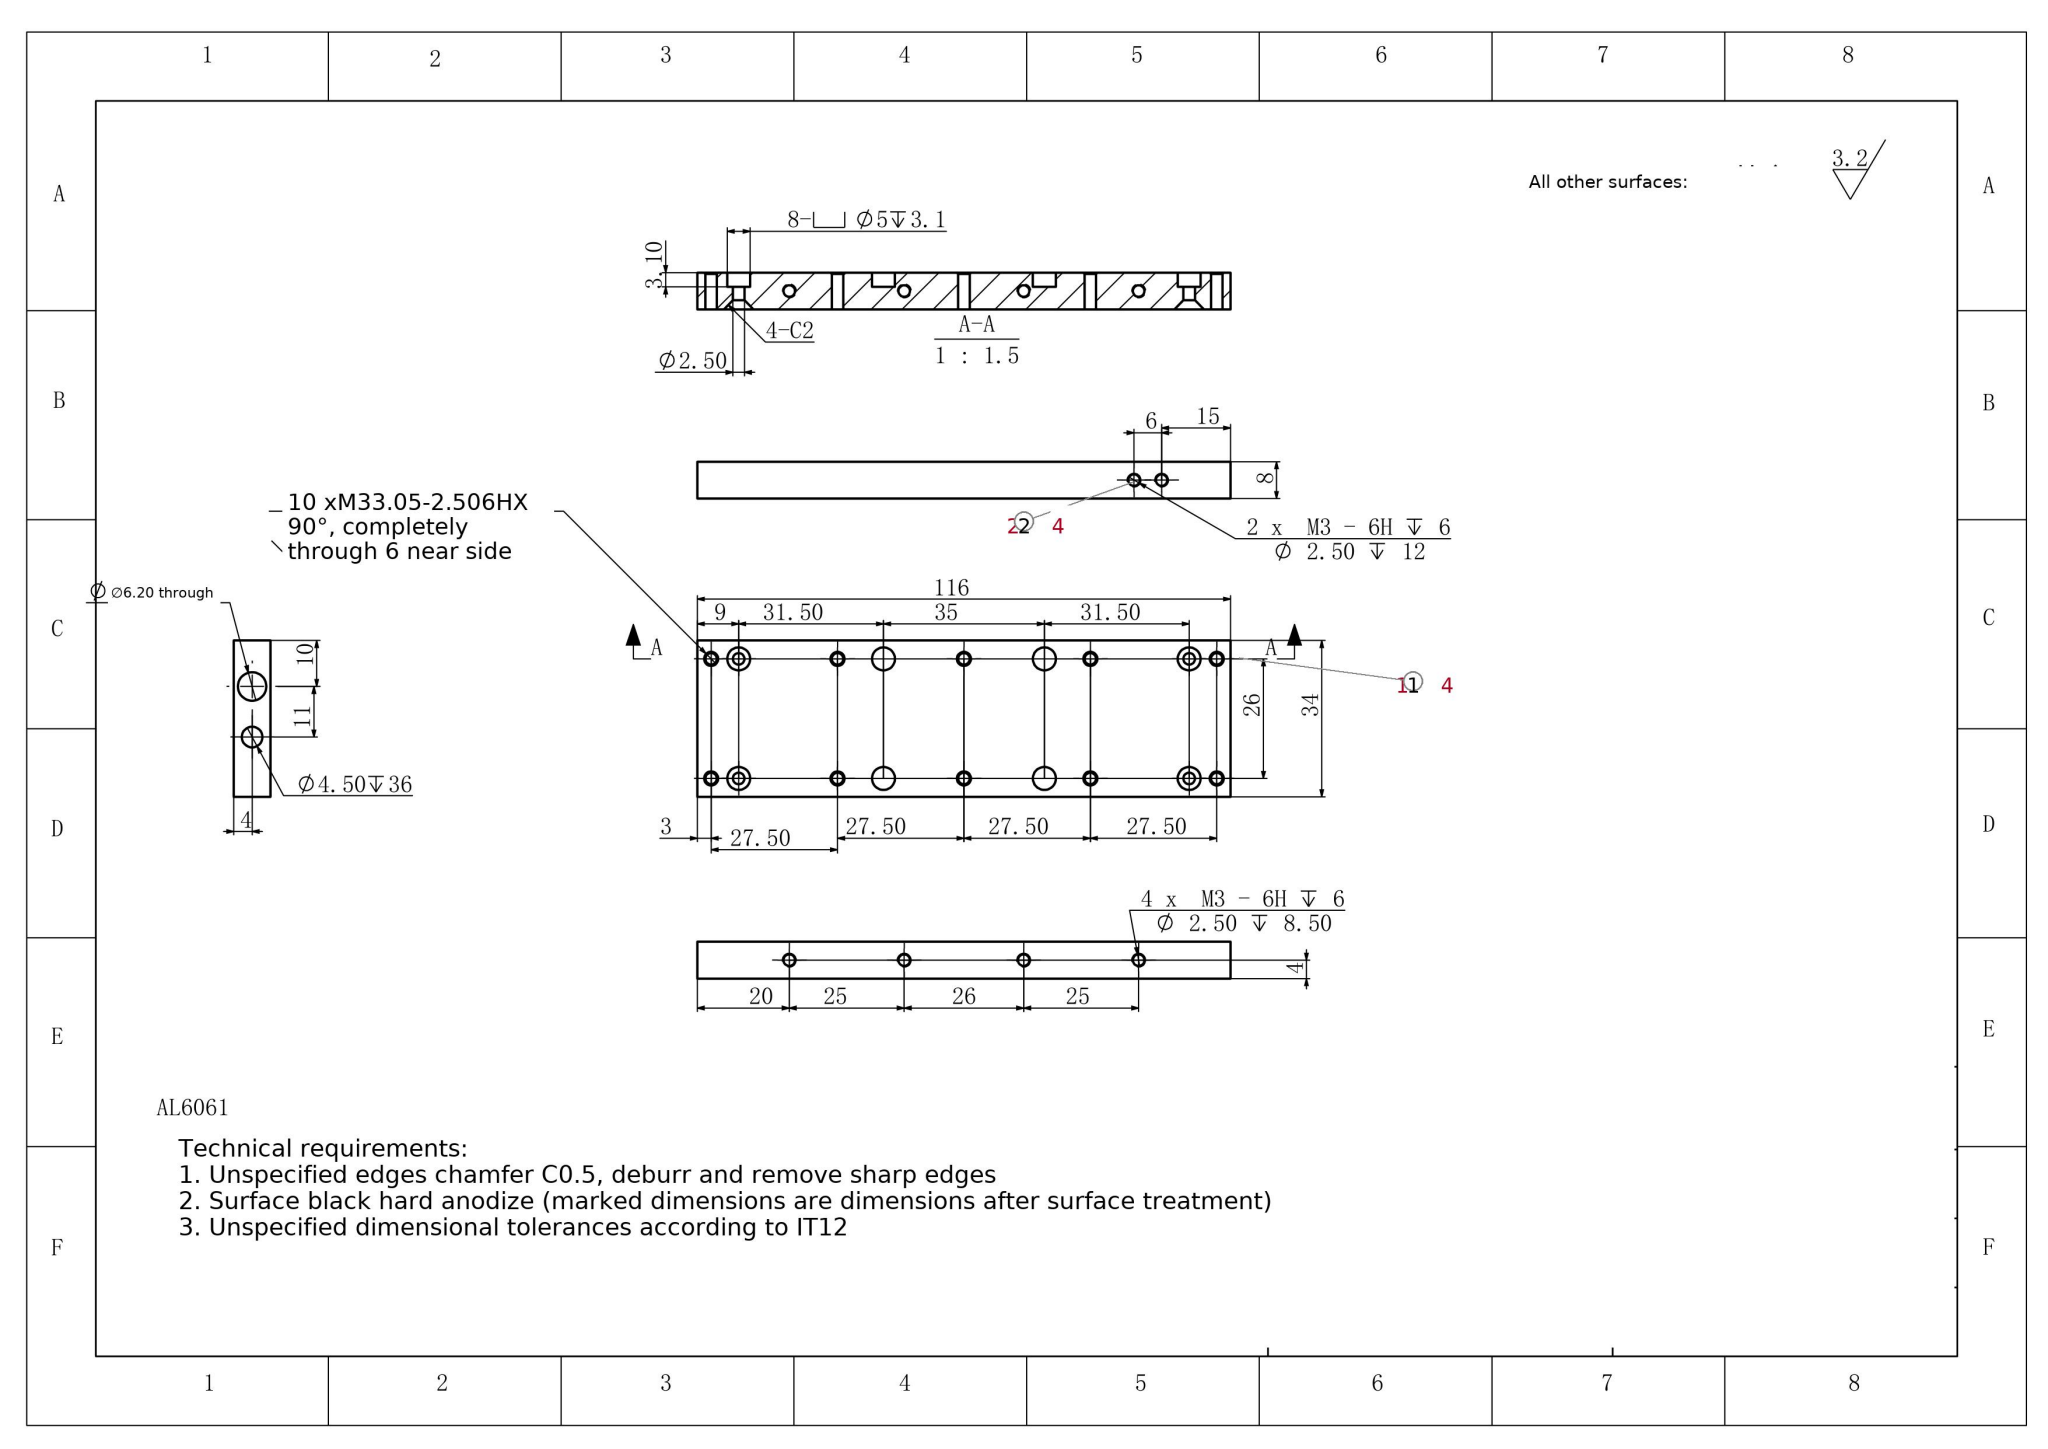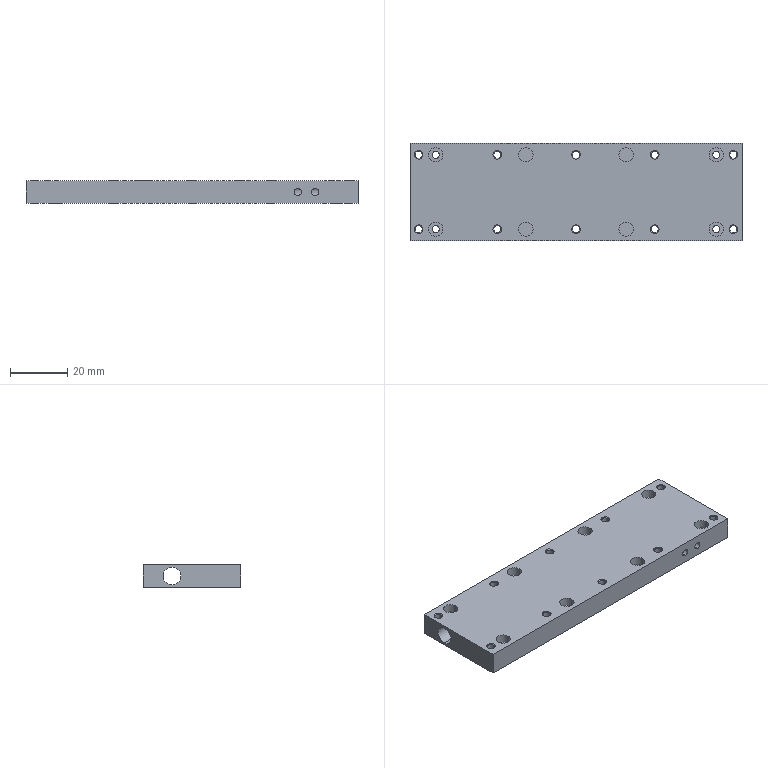Part | SolidWorks | mm | material AL6061 | 1 solid | 103 faces | box 116 x 34 x 8 mm | volume 26159 mm3 | cylinder 60 | cone 28 | plane 15 | commonest cylinder face diameters 2.5 x40 5 x16 4.5 x2 6.2 x2
build123d program:
from build123d import *

# Parameters (mm, degrees)
SKETCH1_W                   = 116
SKETCH1_H                   = 34
BOSS_EXTRUDE1_DEPTH         = 8
F_2_5_2_5_DIAMETER_HOLE1_D  = 2.5
M3_TAPPED_HOLE3_D           = 2.5
M3_TAPPED_HOLE3_CSINK_D     = 3.05
M3_TAPPED_HOLE3_CSINK_ANGLE = 90
SKETCH16_R                  = 3.1
CUT_EXTRUDE2_DEPTH          = 118.512
M3_TAPPED_HOLE5_D           = 2.5
M3_TAPPED_HOLE5_DEPTH       = 8.5
M3_TAPPED_HOLE5_TIP         = 0.7511
SKETCH19_R                  = 2.25
CUT_EXTRUDE3_DEPTH          = 36
M3_TAPPED_HOLE6_D           = 2.5
M3_TAPPED_HOLE6_DEPTH       = 12
M3_TAPPED_HOLE6_TIP         = 0.7511
SKETCH22_R                  = 2.5
CUT_EXTRUDE4_DEPTH          = 3.1
CHAMFER1_SIZE               = 2


with BuildPart() as part:
    # Sketch1 → Boss-Extrude1 (new body)
    with BuildSketch(Plane.XY):
        Rectangle(SKETCH1_W, SKETCH1_H)
    extrude(amount=BOSS_EXTRUDE1_DEPTH)

    # 2.5 _2.5_ Diameter Hole1 (through all)
    with Locations(Plane.XY.offset(8)):
        with Locations((-49, 13), (-49, -13), (49, 13), (49, -13)):
            Hole(F_2_5_2_5_DIAMETER_HOLE1_D / 2)

    # M3 Tapped Hole3 (through all)
    with Locations(Plane.XY.offset(8)):
        with Locations((-55, 13), (-27.5, 13), (0, 13), (27.5, 13), (55, 13), (-55, -13), (-27.5, -13), (0, -13), (27.5, -13), (55, -13)):
            CounterSinkHole(M3_TAPPED_HOLE3_D / 2, M3_TAPPED_HOLE3_CSINK_D / 2, counter_sink_angle=M3_TAPPED_HOLE3_CSINK_ANGLE)

    # Sketch16 → Cut-Extrude2 (cut, through all)
    with BuildSketch(Plane(origin=(58, 0, 0), x_dir=(0, 0, -1), z_dir=(1, 0, 0))):
        with Locations((-4, 7)):
            Circle(SKETCH16_R)
    extrude(amount=-CUT_EXTRUDE2_DEPTH, mode=Mode.SUBTRACT)

    # M3 Tapped Hole5
    with Locations(Plane(origin=(0, 17, 0), x_dir=(1, 0, 0), z_dir=(0, 1, 0))):
        with Locations((38, -4), (-38, -4), (-13, -4), (13, -4)):
            Hole(M3_TAPPED_HOLE5_D / 2, depth=M3_TAPPED_HOLE5_DEPTH)
            with Locations((0, 0, -(M3_TAPPED_HOLE5_DEPTH + M3_TAPPED_HOLE5_TIP / 2))):  # 118° drill point
                Cone(0, M3_TAPPED_HOLE5_D / 2, M3_TAPPED_HOLE5_TIP, mode=Mode.SUBTRACT)

    # Sketch19 → Cut-Extrude3 (cut)
    with BuildSketch(Plane(origin=(58, 0, 0), x_dir=(0, 0, -1), z_dir=(1, 0, 0))):
        with Locations((-4, -4)):
            Circle(SKETCH19_R)
    extrude(amount=-CUT_EXTRUDE3_DEPTH, mode=Mode.SUBTRACT)

    # M3 Tapped Hole6
    with Locations(Plane(origin=(0, -17, 0), x_dir=(-1, 0, 0), z_dir=(0, -1, 0))):
        with Locations((-43, -4), (-37, -4)):
            Hole(M3_TAPPED_HOLE6_D / 2, depth=M3_TAPPED_HOLE6_DEPTH)
            with Locations((0, 0, -(M3_TAPPED_HOLE6_DEPTH + M3_TAPPED_HOLE6_TIP / 2))):  # 118° drill point
                Cone(0, M3_TAPPED_HOLE6_D / 2, M3_TAPPED_HOLE6_TIP, mode=Mode.SUBTRACT)

    # Sketch22 → Cut-Extrude4 (cut)
    with BuildSketch(Plane.XY.offset(8)):
        with Locations((49, 13)):
            Circle(SKETCH22_R)
        with Locations((49, -13)):
            Circle(SKETCH22_R)
        with Locations((-49, -13)):
            Circle(SKETCH22_R)
        with Locations((-49, 13)):
            Circle(SKETCH22_R)
        with Locations((17.5, 13)):
            Circle(SKETCH22_R)
        with Locations((17.5, -13)):
            Circle(SKETCH22_R)
        with Locations((-17.5, 13)):
            Circle(SKETCH22_R)
        with Locations((-17.5, -13)):
            Circle(SKETCH22_R)
    extrude(amount=-CUT_EXTRUDE4_DEPTH, mode=Mode.SUBTRACT)

    # Chamfer1
    chamfer1_edges = [part.edges().sort_by_distance(p)[0] for p in [
        (50.25, -13, 0),
        (50.25, 13, 0),
        (-47.75, -13, 0),
        (-47.75, 13, 0),
    ]]
    chamfer(chamfer1_edges, length=CHAMFER1_SIZE)


solid = part.part